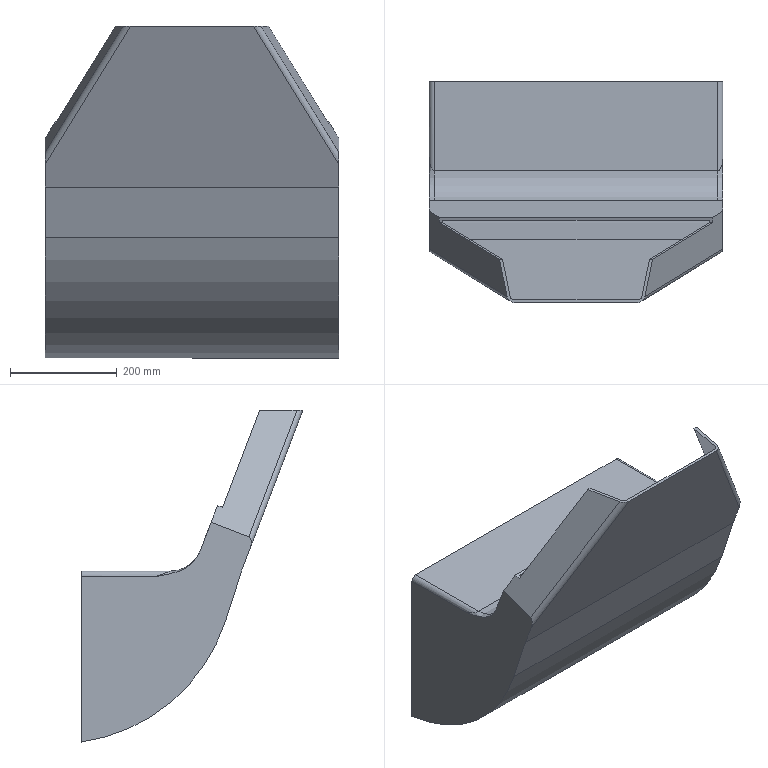Component | SolidWorks | LowerHousing-1 | 1 solid | 37 faces | volume 3791054 mm3 | plane 21 | cylinder 12 | spline 4 | commonest cylinder face diameters 20 x4 10 x4 661.087 x1 651.087 x1 120 x1 130 x1